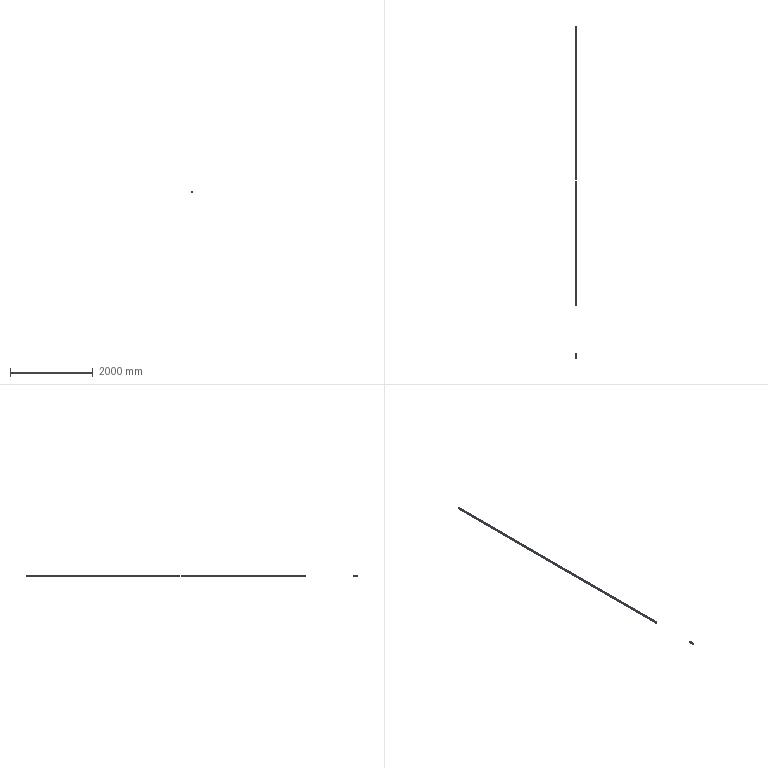Component | SolidWorks | MirrorRailing2-10_Mirror30X30X3-7440-2 | 3 solids | 54 faces | volume 2052415 mm3 | plane 30 | cylinder 24 | commonest cylinder face diameters 6 x12 12 x12